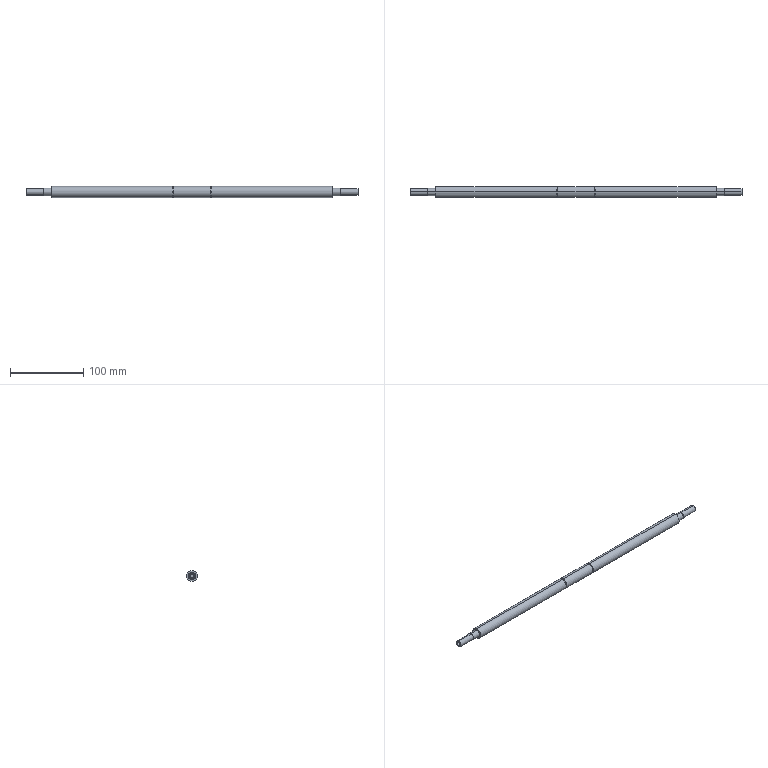Component | SolidWorks | PushRod-1 | 1 solid | 48 faces | volume 71568 mm3 | cylinder 26 | plane 14 | cone 8 | commonest cylinder face diameters 15 x6 5 x4 6 x4 9 x4 10 x4 13 x4